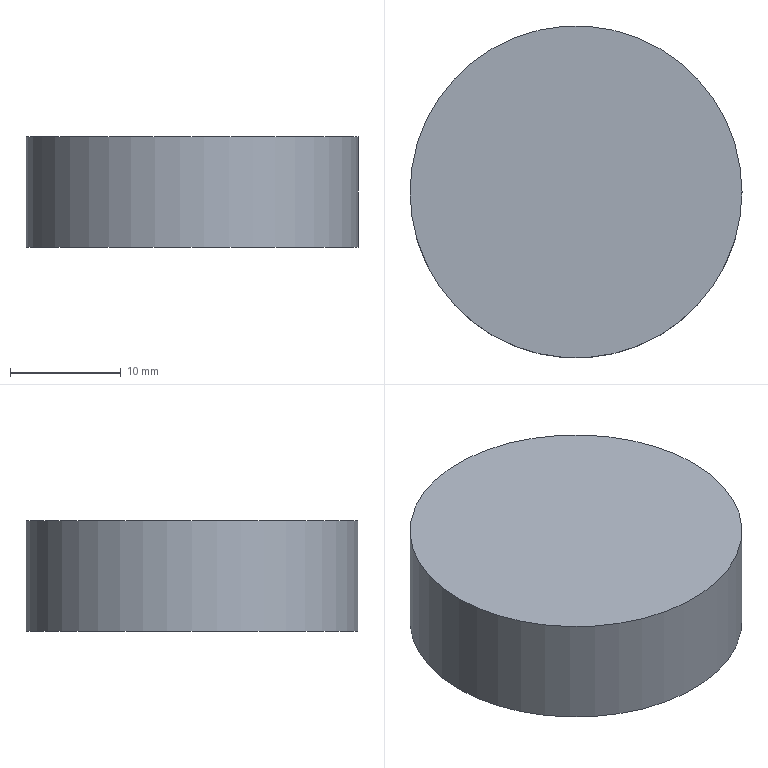Component | NX | CH3404_10-8 | 1 solid | 3 faces | box 30 x 30 x 10 mm | volume 7069 mm3 | plane 2 | cylinder 1 | commonest cylinder face diameters 30 x1
STEP:
#1=CARTESIAN_POINT('',(0.,0.,0.));
#2=DIRECTION('',(0.,0.,1.));
#3=DIRECTION('',(1.,0.,0.));
#4=AXIS2_PLACEMENT_3D('',#1,#2,#3);
#5=CARTESIAN_POINT('',(15.,0.,111.));
#6=VERTEX_POINT('',#5);
#7=CARTESIAN_POINT('',(0.,0.,111.));
#8=DIRECTION('',(0.,0.,1.));
#9=DIRECTION('',(1.,0.,0.));
#10=AXIS2_PLACEMENT_3D('',#7,#8,#9);
#11=CIRCLE('',#10,15.);
#12=CARTESIAN_POINT('',(0.,0.,111.));
#13=DIRECTION('',(0.,0.,-1.));
#14=DIRECTION('',(-1.,0.,0.));
#15=AXIS2_PLACEMENT_3D('',#12,#13,#14);
#16=CYLINDRICAL_SURFACE('',#15,15.);
#17=CARTESIAN_POINT('',(9.425,0.));
#18=DIRECTION('',(-1.,0.));
#19=VECTOR('',#18,1.);
#20=LINE('',#17,#19);
#21=(GEOMETRIC_REPRESENTATION_CONTEXT(2)PARAMETRIC_REPRESENTATION_CONTEXT()REPRESENTATION_CONTEXT('',''));
#22=DEFINITIONAL_REPRESENTATION('',(#20),#21);
#23=PCURVE('',#16,#22);
#24=CARTESIAN_POINT('',(0.,0.,111.));
#25=DIRECTION('',(0.,0.,1.));
#26=DIRECTION('',(1.,0.,0.));
#27=AXIS2_PLACEMENT_3D('',#24,#25,#26);
#28=PLANE('',#27);
#29=CARTESIAN_POINT('',(0.,0.));
#30=DIRECTION('',(1.,0.));
#31=AXIS2_PLACEMENT_2D('',#29,#30);
#32=CIRCLE('',#31,15.);
#33=(GEOMETRIC_REPRESENTATION_CONTEXT(2)PARAMETRIC_REPRESENTATION_CONTEXT()REPRESENTATION_CONTEXT('',''));
#34=DEFINITIONAL_REPRESENTATION('',(#32),#33);
#35=PCURVE('',#28,#34);
#36=SURFACE_CURVE('',#11,(#23,#35),.PCURVE_S1.);
#37=EDGE_CURVE('',#6,#6,#36,.T.);
#38=ORIENTED_EDGE('',*,*,#37,.F.);
#39=CARTESIAN_POINT('',(15.,0.,101.));
#40=VERTEX_POINT('',#39);
#41=CARTESIAN_POINT('',(15.,0.,111.));
#42=CARTESIAN_POINT('',(15.,0.,101.));
#43=B_SPLINE_CURVE_WITH_KNOTS('',1,(#41,#42),.UNSPECIFIED.,.F.,.F.,(2,2),(0.,10.),.PIECEWISE_BEZIER_KNOTS.);
#44=CARTESIAN_POINT('',(9.425,0.));
#45=DIRECTION('',(0.,1.));
#46=VECTOR('',#45,1.);
#47=LINE('',#44,#46);
#48=(GEOMETRIC_REPRESENTATION_CONTEXT(2)PARAMETRIC_REPRESENTATION_CONTEXT()REPRESENTATION_CONTEXT('',''));
#49=DEFINITIONAL_REPRESENTATION('',(#47),#48);
#50=PCURVE('',#16,#49);
#51=CARTESIAN_POINT('',(3.142,0.));
#52=DIRECTION('',(0.,1.));
#53=VECTOR('',#52,1.);
#54=LINE('',#51,#53);
#55=(GEOMETRIC_REPRESENTATION_CONTEXT(2)PARAMETRIC_REPRESENTATION_CONTEXT()REPRESENTATION_CONTEXT('',''));
#56=DEFINITIONAL_REPRESENTATION('',(#54),#55);
#57=PCURVE('',#16,#56);
#58=SEAM_CURVE('',#43,(#50,#57),.PCURVE_S1.);
#59=EDGE_CURVE('',#6,#40,#58,.T.);
#60=ORIENTED_EDGE('',*,*,#59,.T.);
#61=CARTESIAN_POINT('',(0.,0.,101.));
#62=DIRECTION('',(0.,0.,1.));
#63=DIRECTION('',(1.,0.,0.));
#64=AXIS2_PLACEMENT_3D('',#61,#62,#63);
#65=CIRCLE('',#64,15.);
#66=CARTESIAN_POINT('',(9.425,10.));
#67=DIRECTION('',(-1.,0.));
#68=VECTOR('',#67,1.);
#69=LINE('',#66,#68);
#70=(GEOMETRIC_REPRESENTATION_CONTEXT(2)PARAMETRIC_REPRESENTATION_CONTEXT()REPRESENTATION_CONTEXT('',''));
#71=DEFINITIONAL_REPRESENTATION('',(#69),#70);
#72=PCURVE('',#16,#71);
#73=CARTESIAN_POINT('',(0.,0.,101.));
#74=DIRECTION('',(0.,0.,1.));
#75=DIRECTION('',(1.,0.,0.));
#76=AXIS2_PLACEMENT_3D('',#73,#74,#75);
#77=PLANE('',#76);
#78=CARTESIAN_POINT('',(0.,0.));
#79=DIRECTION('',(1.,0.));
#80=AXIS2_PLACEMENT_2D('',#78,#79);
#81=CIRCLE('',#80,15.);
#82=(GEOMETRIC_REPRESENTATION_CONTEXT(2)PARAMETRIC_REPRESENTATION_CONTEXT()REPRESENTATION_CONTEXT('',''));
#83=DEFINITIONAL_REPRESENTATION('',(#81),#82);
#84=PCURVE('',#77,#83);
#85=SURFACE_CURVE('',#65,(#72,#84),.PCURVE_S1.);
#86=EDGE_CURVE('',#40,#40,#85,.T.);
#87=ORIENTED_EDGE('',*,*,#86,.T.);
#88=ORIENTED_EDGE('',*,*,#59,.F.);
#89=EDGE_LOOP('',(#38,#60,#87,#88));
#90=FACE_BOUND('',#89,.T.);
#91=ADVANCED_FACE('',(#90),#16,.T.);
#92=ORIENTED_EDGE('',*,*,#37,.T.);
#93=EDGE_LOOP('',(#92));
#94=FACE_BOUND('',#93,.T.);
#95=ADVANCED_FACE('',(#94),#28,.T.);
#96=ORIENTED_EDGE('',*,*,#86,.F.);
#97=EDGE_LOOP('',(#96));
#98=FACE_BOUND('',#97,.T.);
#99=ADVANCED_FACE('',(#98),#77,.F.);
#100=CLOSED_SHELL('',(#91,#95,#99));
#101=MANIFOLD_SOLID_BREP('',#100);
#102=(LENGTH_UNIT()NAMED_UNIT(*)SI_UNIT(.MILLI.,.METRE.));
#103=UNCERTAINTY_MEASURE_WITH_UNIT(LENGTH_MEASURE(0.00001),#102,'','');
#104=(NAMED_UNIT(*)PLANE_ANGLE_UNIT()SI_UNIT($,.RADIAN.));
#105=(NAMED_UNIT(*)SI_UNIT($,.STERADIAN.)SOLID_ANGLE_UNIT());
#106=(GEOMETRIC_REPRESENTATION_CONTEXT(3)GLOBAL_UNCERTAINTY_ASSIGNED_CONTEXT((#103))GLOBAL_UNIT_ASSIGNED_CONTEXT((#102,#104,#105))REPRESENTATION_CONTEXT('',''));
#107=ADVANCED_BREP_SHAPE_REPRESENTATION('',(#4,#101),#106);